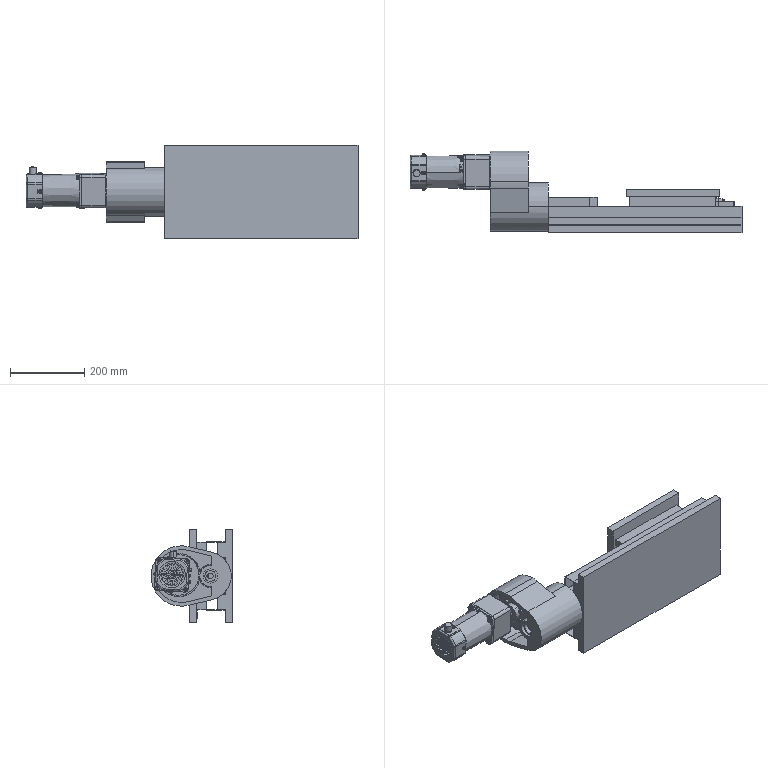Assembly | SolidWorks | mm | 44 component files | 283 solids | 3071 faces | box 892.1 x 219.71 x 250 mm | volume 9592429 mm3 | cylinder 1011 | sphere 848 | plane 709 | spline 244 | cone 147 | torus 112 | commonest cylinder face diameters 115.5 x76 108.75 x75 2 x53 20 x52 15 x47 39 x38 50.25 x36 57 x36
Bill of materials:
BallScrew | 1 |  | Long, slender, round stepped shaft. It has a band of evenly spaced circumferential grooves partway along its length, and both ends step down to smaller diameters.
BearingHousing | 1 |  | Two separate prismatic bodies: a thick rectangular plate with a large round through-hole, and a near-cubic block with a small rectangular through-opening.
ConnectingFlange | 2 |  | Long, thin-walled formed or extruded profile with a constant cross-section that has several 90-degree bends.
ConnectingSeat | 1 |  | Rectangular block with a large round through-bore and a taller flange-like section along one side, giving a stepped end profile.
CopperGasket | 1 |  | Two separate thin flat plates: a rectangular plate with four small holes near its corners, and a long narrow plain strip.
CountersunkScrewM5X20 | 6 |  | Stepped cylindrical pin with a larger-diameter head and a smaller shank. The head end face has a polygonal recess, and the shank tip is chamfered.
CountersunkScrewM8x4 | 4 |  | Stepped cylindrical pin with a larger cylindrical head and a smaller, longer shank with a chamfered tip.
CouplingSleeve | 1 |  | Thick-walled cylindrical sleeve with a round bore and two rectangular keyway-like notches cut into the bore.
DeepGrooveBallBearing16002 | 5 |  | Annular ring assembly that looks like a rolling-element bearing: outer ring, wide inner ring with a moderate bore, and a single row of balls between them.
DeepGrooveBallBearing6204 | 1 |  | Thin-section annular ring assembly that looks like a rolling-element bearing: narrow outer and inner rings, a large bore, and a single row of balls.
EndCap | 1 |  | Bracket-like part: a flat rectangular plate with four holes, two near each end, and a hollow rectangular frame or tube sticking out from one face.
GearAxis | 1 |  | Long, solid, round rod with a small flat or notch cut at one end and a slight step near the other end.
Gearbox | 1 |  | Solid with a pear/cam-shaped outline: a large circular lobe and a smaller circular lobe joined by tangent flat sides. The two lobes have different axial lengths, which makes a step in the side views. There is a through hole in the smaller lobe.
HexSocketScrewM6X15 | 1 |  | Cap-screw-like solid: a cylindrical head with a hexagonal socket recess, and a long plain cylindrical shank with a chamfered end.
NutSeat | 1 |  | Rectangular block with one round hole through one face; the hole sits off-center.
OilCup | 1 |  | Stepped turned part with a hexagonal flange: a short cylindrical collar on one side of the hex, then a larger cylindrical body, a smaller chamfered step, and a small cylindrical tip ending in a cone.
OriginalWasher | 2 |  | Thin-walled cylindrical ring with a narrow radial wall and short axial length.
ParallelKey5x5x25 | 1 |  | Obround (slot-shaped) prism: a straight bar with fully rounded ends and flat parallel top and bottom faces.
ReducerLargeGear | 1 |  | Large spur-type gear with many straight teeth, a central bore, six evenly spaced round holes in the web, and a cylindrical hub on one face.
ReducerSmallGear | 1 |  | Small spur-type gear (pinion-like) with straight teeth, a central round bore, and a cylindrical hub on one side.
RoundNut | 2 |  | Thick flat annular ring (washer or spacer shape) with plain cylindrical inner and outer surfaces.
RoundNutLockingWasher15 | 2 |  | Thin annular disc with a conical (dished) form. The side profile is a slanted parallelogram, and the outer edge looks beveled.
SealingAnvil | 1 |  | Flat plate of constant thickness with a T-like outline: a long rectangular bar with a wider rectangular tab off one side, and one round through hole in the tab.
SealingFelt | 1 |  | Annular washer-like disc with a central hole and chamfered outer edges on both faces, so the side profile looks like a symmetric flattened hexagon.
ShaftRetainingRing | 1 |  | Flat annular ring (plain washer-like disc): thin circular disc with a concentric circular through hole.
StepperMotor | 1 |  | Elongated motor-like unit: a cylindrical main body with a rounded end cap at one end and a square housing at the other end. A cylindrical output shaft sticks out from the centre of the square end face.
WorkPlatform | 1 |  | Square flat plate with two parallel rectangular rails raised on one face, and a small pattern of holes in the plain area between or beside the rails.
X-AxisSupportBase | 1 |  | Thin rectangular plate whose cross-section is stepped along one face. Two rectangular ribs and a slightly lower central raised land are separated by narrow gaps.
Mates:
1. parallel | X-AxisSupportBase-1 face at (0, 40, 90.896) dir (0, 0, 1) | ConnectingFlange-3 face at (-277, 70, 90.896) dir (0, 0, -1)
2. parallel | X-AxisSupportBase-1 face at (-277, 20, 115) dir (-1, 0, 0) | ConnectingFlange-3 face at (-277, 70, 91.632) dir (-1, 0, 0)
3. coincident | X-AxisSupportBase-1 face at (-277, 20, 115) dir (-1, 0, 0) | ConnectingFlange-3 face at (-277, 70, 48.661) dir (-1, 0, 0)
4. coincident | X-AxisSupportBase-1 face at (0, 20, 0) dir (0, 1, 0) | ConnectingFlange-3 face at (0, 20, 0) dir (0, -1, 0)
5. coincident | X-AxisSupportBase-1 face at (503, 0, 49.398) dir (0, 0, -1) | ConnectingFlange-3 face at (0, 20, 49.398) dir (0, 0, 1)
6. parallel | X-AxisSupportBase-1 face at (0, 0, 0) dir (0, -1, 0) | WorkPlatform-1 face at (56.772, 116.74, 0) dir (0, 1, 0)
7. parallel | X-AxisSupportBase-1 face at (-277, 20, 115) dir (0, 0, 1) | WorkPlatform-1 face at (171.772, 116.74, 115) dir (0, 0, 1)
8. coincident | X-AxisSupportBase-1 face at (0, 20, 0) dir (0, 1, 0) | ConnectingSeat-1 face at (-166, 20, 46.072) dir (0, -1, 0)
9. coincident | X-AxisSupportBase-1 face at (-277, 20, 115) dir (-1, 0, 0) | ConnectingSeat-1 face at (-277, 40, 0) dir (-1, 0, 0)
10. coincident | ConnectingSeat-1 face at (-277, 40, 0) dir (-1, 0, 0) | Gearbox-1 face at (-277, 69.2, 0) dir (1, 0, 0)
11. concentric | Gearbox-1 face at (-302, 60.219, 0) dir (1, 0, 0) r 25.57 | ReducerSmallGear-1 face at (-323.574, 60.219, 0) dir (-1, 0, 0) r 7.5
12. coincident | Gearbox-1 plane at (-277, 0, 0) dir (0, 0, -1) | assembly plane at (0, 0, 0) dir (0, 0, 1)
13. concentric | BallScrew-1 face at (263, 60.219, 0) dir (1, 0, 0) r 7.5 | BearingHousing-1 face at (194.019, 60.219, 0) dir (-1, 0, 0) r 10.5
14. coincident | BearingHousing-1 face at (178.784, 85.587, 21.161) dir (-1, 0, 0) | EndCap-2 face at (178.784, 77.114, 0) dir (1, 0, 0)
15. coincident | BearingHousing-1 face at (-54.961, 84.114, 27.5) dir (0, 1, 0) | EndCap-2 face at (158.784, 84.114, -27.5) dir (0, 1, 0)
16. coincident | BearingHousing-1 face at (-54.961, 85.587, 27.5) dir (0, 0, 1) | EndCap-2 face at (158.784, 84.114, 27.5) dir (0, 0, 1)
17. concentric | BallScrew-1 face at (263, 60.219, 0) dir (-1, 0, 0) r 10 | NutSeat-1 face at (-31.284, 60.219, 0) dir (1, 0, 0) r 10
18. coincident | BallScrew-1 sketch segment at (103, 60.219, 0) dir (1, 0, 0) r 10 | NutSeat-1 sketch segment at (103, 60.219, 0) dir (1, 0, 0) r 10
19. concentric | ConnectingSeat-1 face at (-281, 60.219, 0) dir (1, 0, 0) r 25.57 | DeepGrooveBallBearing16002-1 face at (-186, 60.219, 0) dir (-1, 0, 0) r 23.5
20. coincident | ConnectingSeat-1 face at (-166, 40, 0) dir (1, 0, 0) | DeepGrooveBallBearing16002-2 face at (-166, 82.472, 6.559) dir (1, 0, 0)
21. concentric | BallScrew-1 face at (-250, 60.219, 0) dir (1, 0, 0) r 6.215 | CouplingSleeve-1 face at (-286.5, 60.219, 0) dir (1, 0, 0) r 8.58
22. distance | GearAxis-1 face at (-277, 60.219, 0) dir (1, 0, 0) | BallScrew-1 face at (-272, 60.219, 0) dir (-1, 0, 0)
23. coincident | ReducerSmallGear-1 face at (-413, 60.219, 0) dir (-1, 0, 0) | GearAxis-1 face at (-413, 60.219, 0) dir (-1, 0, 0)
24. coincident | GearAxis-1 face at (-282, 57.736, 2.456) dir (0, 0.9986, -0.05333) | ParallelKey5x5x25-1 face at (-14.748, 58.109, 9.447) dir (0, -0.9986, 0.05333)
25. coincident | BallScrew-1 face at (-265, 57.736, 2.456) dir (0, 0.9986, -0.05333) | ParallelKey5x5x25-1 face at (-14.748, 58.109, 9.447) dir (0, -0.9986, 0.05333)
26. coincident | GearAxis-1 face at (-282, 57.736, 2.456) dir (0, 0.05333, 0.9986) | ParallelKey5x5x25-1 edge at (-280.428, 57.736, 2.456) dir (1, 0, 0)
27. coincident | BallScrew-1 face at (-265, 57.736, 2.456) dir (0, 0.05333, 0.9986) | ParallelKey5x5x25-1 edge at (-280.428, 57.736, 2.456) dir (1, 0, 0)
28. tangent | GearAxis-1 face at (-282, 57.007, -60.133) dir (1, 0, 0) | ParallelKey5x5x25-1 face at (-279.134, 60.289, 2.32) dir (0, 0.05333, 0.9986) r 2.866
29. concentric | BallScrew-1 face at (-250, 60.219, 0) dir (1, 0, 0) r 6.215 | Gearbox-1 face at (-292, 60.219, 0) dir (1, 0, 0) r 18.564
30. concentric | Gearbox-1 face at (-398.993, 60.219, 0) dir (-1, 0, 0) r 15 | GearAxis-1 edge at (-413, 60.219, 0) dir (-1, 0, 0) r 7.5
31. coincident | BallScrew-1 edge at (-249.5, 60.219, 0) dir (1, 0, 0) r 6.215 | CouplingSleeve-1 face at (-249.5, 60.219, 0) dir (1, 0, 0)
32. concentric | BallScrew-1 face at (263, 60.219, 0) dir (-1, 0, 0) r 10 | RoundNutLockingWasher15-1 edge at (-186, 60.219, 0) dir (-1, 0, 0) r 10.006
33. concentric | BallScrew-1 face at (263, 60.219, 0) dir (-1, 0, 0) r 10 | RoundNut-1 face at (-196.75, 60.219, 0) dir (1, 0, 0) r 19.5
34. coincident | RoundNut-1 edge at (-187.75, 60.219, 0) dir (-1, 0, 0) r 19.5 | RoundNutLockingWasher15-1 edge at (-187.75, 60.219, 0) dir (-1, 0, 0) r 19.5
35. coincident | DeepGrooveBallBearing16002-1 face at (-186, 52.87, -16.212) dir (-1, 0, 0) | RoundNutLockingWasher15-1 face at (-186, 80.498, 0) dir (1, 0, 0)
36. coincident | DeepGrooveBallBearing16002-1 face at (-179, 52.168, -17.76) dir (1, 0, 0) | OriginalWasher-1 face at (-179, 59.486, -0.1318) dir (-1, 0, 0)
37. coincident | DeepGrooveBallBearing16002-2 face at (-173, 77.293, 5.033) dir (-1, 0, 0) | OriginalWasher-1 face at (-173, 59.486, -0.1318) dir (1, 0, 0)
38. concentric | BallScrew-1 face at (263, 60.219, 0) dir (-1, 0, 0) r 10 | OriginalWasher-1 face at (-176, 60.219, 0) dir (1, 0, 0) r 16.311
39. coincident | Gearbox-1 face at (-331, 60.219, 0) dir (-1, 0, 0) | DeepGrooveBallBearing16002-4 face at (-331, 83.419, 0) dir (-1, 0, 0)
40. concentric | BallScrew-1 face at (263, 60.219, 0) dir (-1, 0, 0) r 10 | SealingAnvil-1 face at (-146, 60.219, 0) dir (-1, 0, 0) r 10
41. parallel | X-AxisSupportBase-1 face at (0, 20, 0) dir (0, 1, 0) | SealingAnvil-1 face at (-146, 39.822, -46.072) dir (0, 1, 0)
42. coincident | X-AxisSupportBase-1 face at (0, 20, 0) dir (0, 1, 0) | SealingAnvil-1 edge at (-166, 20, 46.072) dir (0, 0, -1)
43. coincident | ConnectingSeat-1 face at (-166, 40, 0) dir (1, 0, 0) | SealingAnvil-1 face at (-166, 0, 0) dir (-1, 0, 0)
44. concentric | BallScrew-1 face at (263, 60.219, 0) dir (-1, 0, 0) r 10 | DeepGrooveBallBearing16002-5 face at (236.13, 60.219, 0) dir (-1, 0, 0) r 11.01
45. coincident | EndCap-2 face at (178.784, 77.114, 0) dir (1, 0, 0) | DeepGrooveBallBearing16002-5 face at (178.784, 67.423, 22.053) dir (-1, 0, 0)
46. concentric | BallScrew-1 face at (263, 60.219, 0) dir (1, 0, 0) r 7.5 | DeepGrooveBallBearing16002-6 face at (249.13, 60.219, 0) dir (-1, 0, 0) r 11.01
47. concentric | BallScrew-1 face at (263, 60.219, 0) dir (1, 0, 0) r 7.5 | OriginalWasher-2 face at (188.784, 60.219, 0) dir (1, 0, 0) r 19.557
48. coincident | DeepGrooveBallBearing16002-5 face at (185.784, 66.274, 18.536) dir (1, 0, 0) | OriginalWasher-2 face at (185.784, 59.486, -0.1289) dir (-1, 0, 0)
49. coincident | DeepGrooveBallBearing16002-6 face at (191.784, 74.631, 10.446) dir (-1, 0, 0) | OriginalWasher-2 face at (191.784, 59.486, -0.1289) dir (1, 0, 0)
50. coincident | DeepGrooveBallBearing16002-6 face at (198.784, 76.008, 11.444) dir (1, 0, 0) | RoundNutLockingWasher15-2 face at (198.784, 63.32, 20.04) dir (-1, 0, 0)
51. concentric | RoundNutLockingWasher15-2 edge at (200.384, 60.219, 0) dir (1, 0, 0) r 10.006 | RoundNut-2 face at (200.534, 60.219, 0) dir (1, 0, 0) r 10
52. coincident | RoundNutLockingWasher15-2 face at (200.534, 60.219, 0) dir (-1, 0, 0) r 1554.999 | RoundNut-2 edge at (200.534, 60.219, 0) dir (-1, 0, 0) r 19.5
53. concentric | Gearbox-1 face at (-425, 60.219, 0) dir (-1, 0, 0) r 19.092 | DeepGrooveBallBearing6204-2 face at (-413, 60.219, 0) dir (-1, 0, 0) r 15
54. coincident | Gearbox-1 face at (-406, 60.219, 0) dir (1, 0, 0) | DeepGrooveBallBearing6204-2 face at (-406, 80.67, -3.201) dir (1, 0, 0)
55. parallel | ReducerSmallGear-1 face at (-396, 59.531, 2.626) dir (0, 0.2533, -0.9674) | GearAxis-1 face at (-388.806, 41.788, -2.021) dir (0, 0.2533, -0.9674)
56. coincident | ReducerSmallGear-1 face at (-366, 60.219, 0) dir (1, 0, 0) | ShaftRetainingRing-1 edge at (-366, 60.219, 0) dir (1, 0, 0) r 15.026
57. coincident | ReducerSmallGear-1 face at (-413, 60.219, 0) dir (-1, 0, 0) | DeepGrooveBallBearing6204-2 edge at (-413, 60.219, 0) dir (-1, 0, 0) r 15.3
58. parallel | ReducerSmallGear-1 face at (-413, 60.219, 0) dir (-1, 0, 0) | ReducerLargeGear-4 face at (-410, 145.203, 2.782) dir (-1, 0, 0)
59. concentric | StepperMotor-2 face at (-426.5, 145.203, 2.782) dir (1, 0, 0) r 7.5 | ReducerLargeGear-4 face at (-318, 145.203, 2.782) dir (-1, 0, 0) r 14.069
60. coincident | Gearbox-1 face at (-434, 138.635, 0) dir (-1, 0, 0) | StepperMotor-2 face at (-434, 163.177, 3.733) dir (1, 0, 0)
61. coincident | ReducerLargeGear-4 face at (-376, 115.174, 16.323) dir (1, 0, 0) | CountersunkScrewM5X20-1 edge at (-376, 115.174, 16.323) dir (1, 0, 0) r 7.5
62. concentric | ReducerLargeGear-4 face at (-376, 115.174, 16.323) dir (1, 0, 0) r 7.5 | CountersunkScrewM5X20-1 face at (-362, 115.174, 16.323) dir (-1, 0, 0) r 7.5
63. coincident | WorkPlatform-1 face at (56.772, 96.74, 0) dir (0, -1, 0) | CopperGasket-1 face at (-3, 96.74, 0) dir (0, 1, 0)
64. concentric | WorkPlatform-1 face at (86.571, 106.74, -20.473) dir (0, 1, 0) r 4.017 | CountersunkScrewM8x4-2 face at (86.571, 87.74, -20.473) dir (0, 1, 0) r 2.271
65. concentric | WorkPlatform-1 face at (86.571, 58.74, 20.473) dir (0, 1, 0) r 2.271 | CountersunkScrewM8x4-4 face at (86.571, 87.74, 20.473) dir (0, 1, 0) r 2.271
66. concentric | WorkPlatform-1 face at (26.973, 58.74, 20.473) dir (0, 1, 0) r 2.271 | CountersunkScrewM8x4-3 face at (26.973, 87.74, 20.473) dir (0, 1, 0) r 2.271
67. coincident | ReducerSmallGear-1 face at (-396, 60.219, 0) dir (-1, 0, 0) | ReducerLargeGear-4 face at (-396, 145.203, 2.782) dir (-1, 0, 0)
68. gear | ReducerSmallGear-1 sketch segment at (-396, 60.219, 0) dir (-1, 0, 0) r 26.846 | ReducerLargeGear-4 sketch segment at (-396, 145.203, 2.782) dir (-1, 0, 0) r 56.581
69. concentric | WorkPlatform-1 face at (167.772, 84.115, -69.517) dir (1, 0, 0) r 9.38 | OilCup-2 edge at (169.772, 84.115, -69.517) dir (1, 0, 0) r 8.316
70. coincident | WorkPlatform-1 face at (171.772, 116.74, 115) dir (1, 0, 0) | OilCup-2 edge at (171.772, 76.733, -77.511) dir (0, 0.9755, -0.2202)
71. parallel | X-AxisSupportBase-1 face at (0, 40, 0) dir (0, 1, 0) | BearingHousing-1 face at (-54.961, 84.114, 27.5) dir (0, 1, 0)